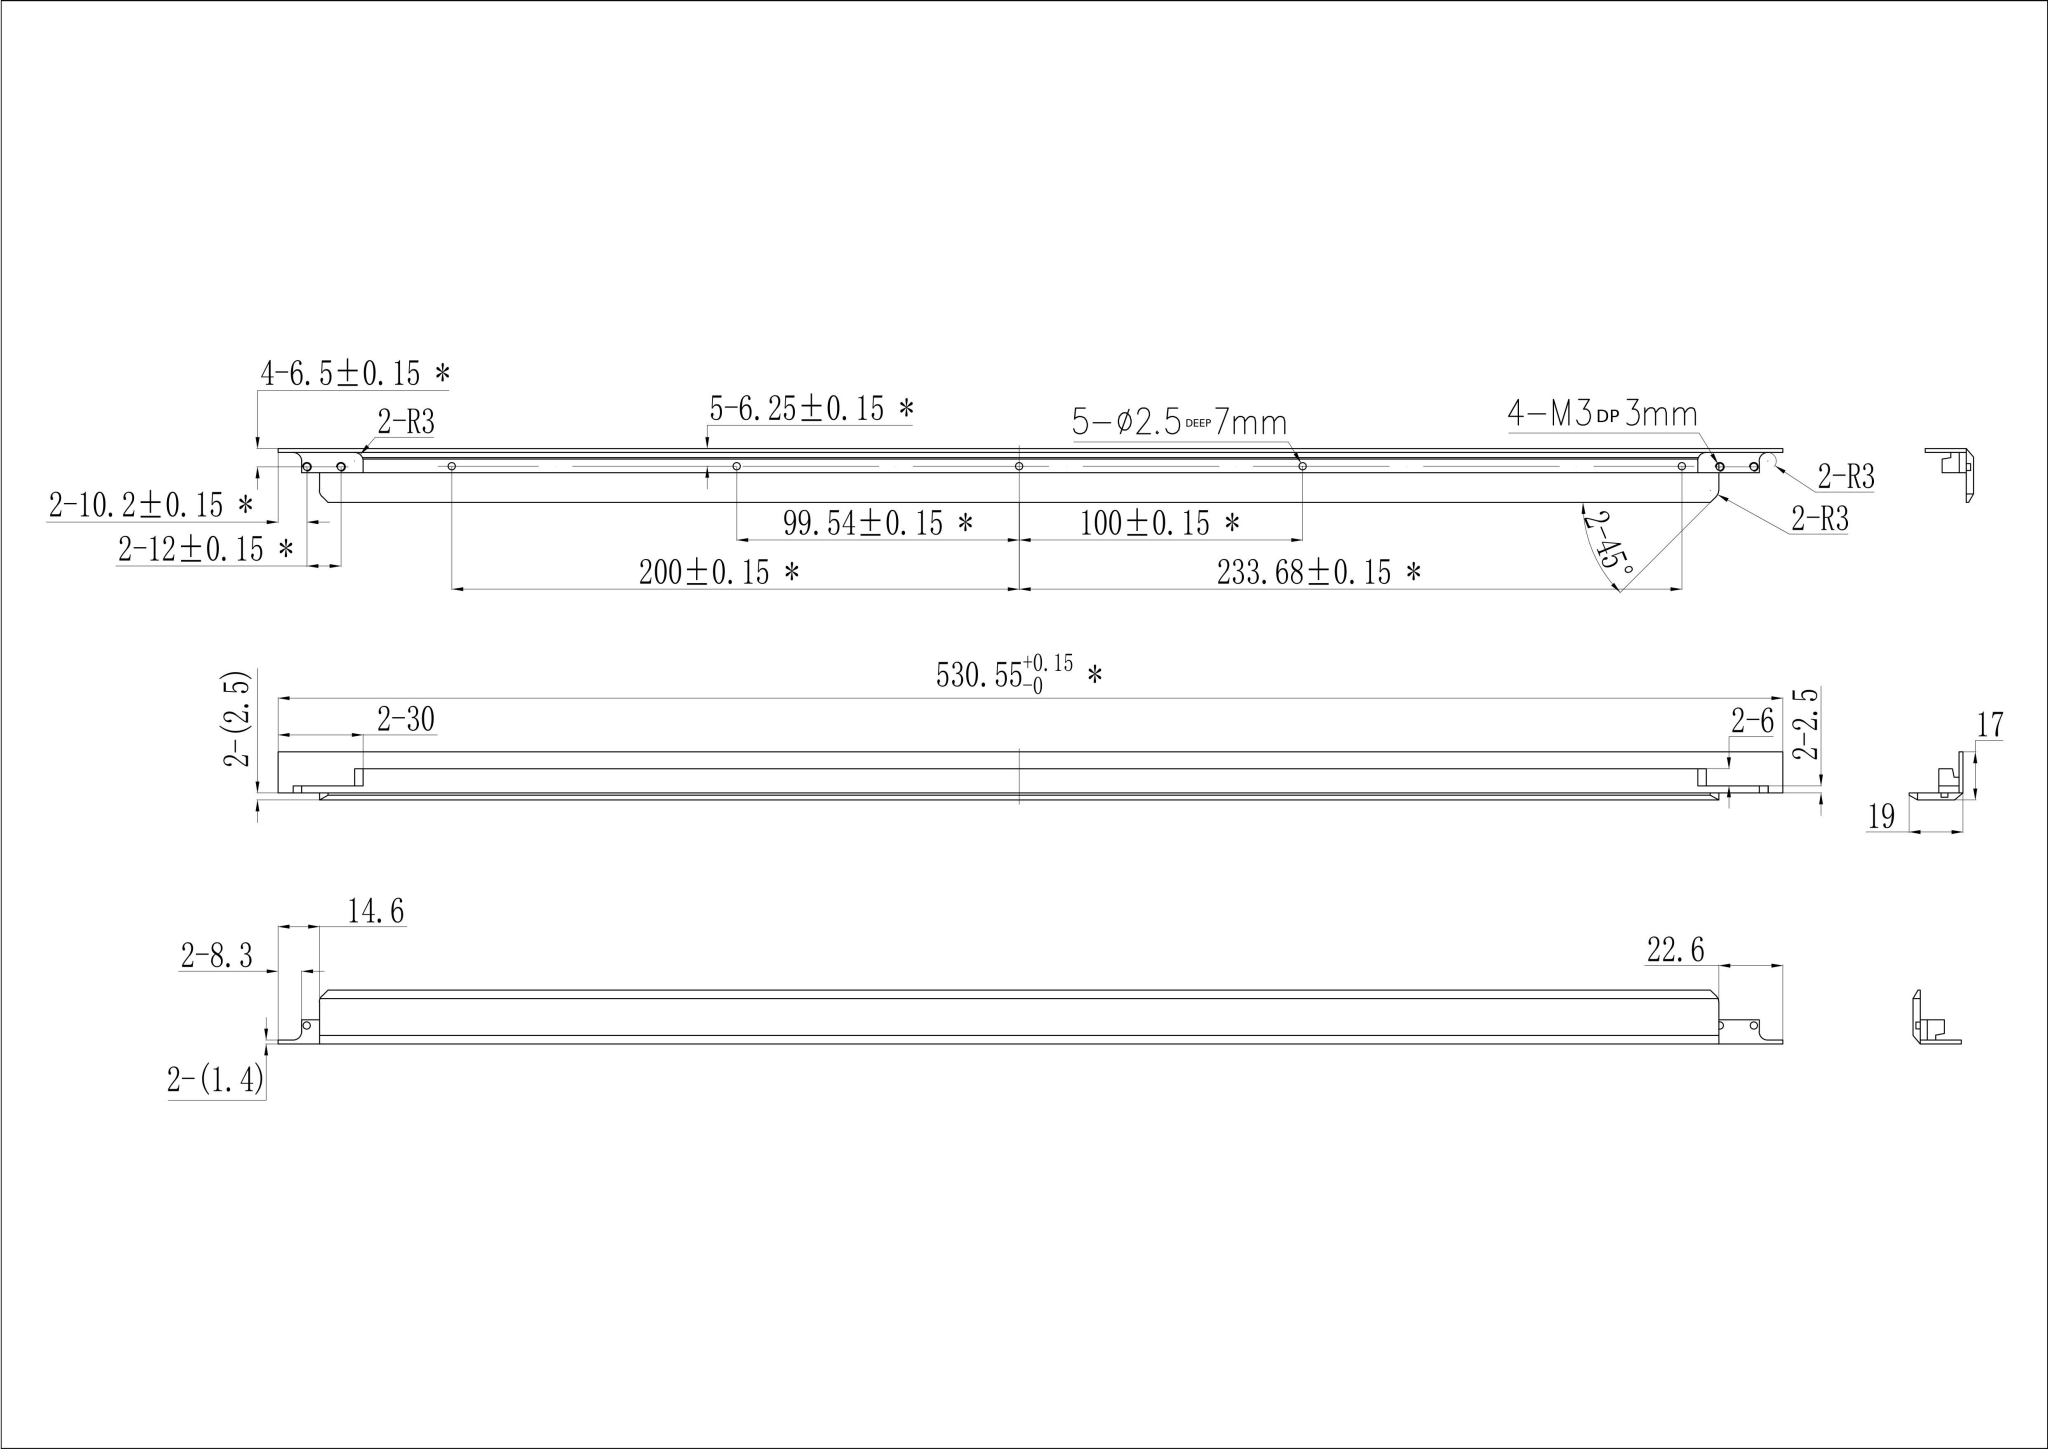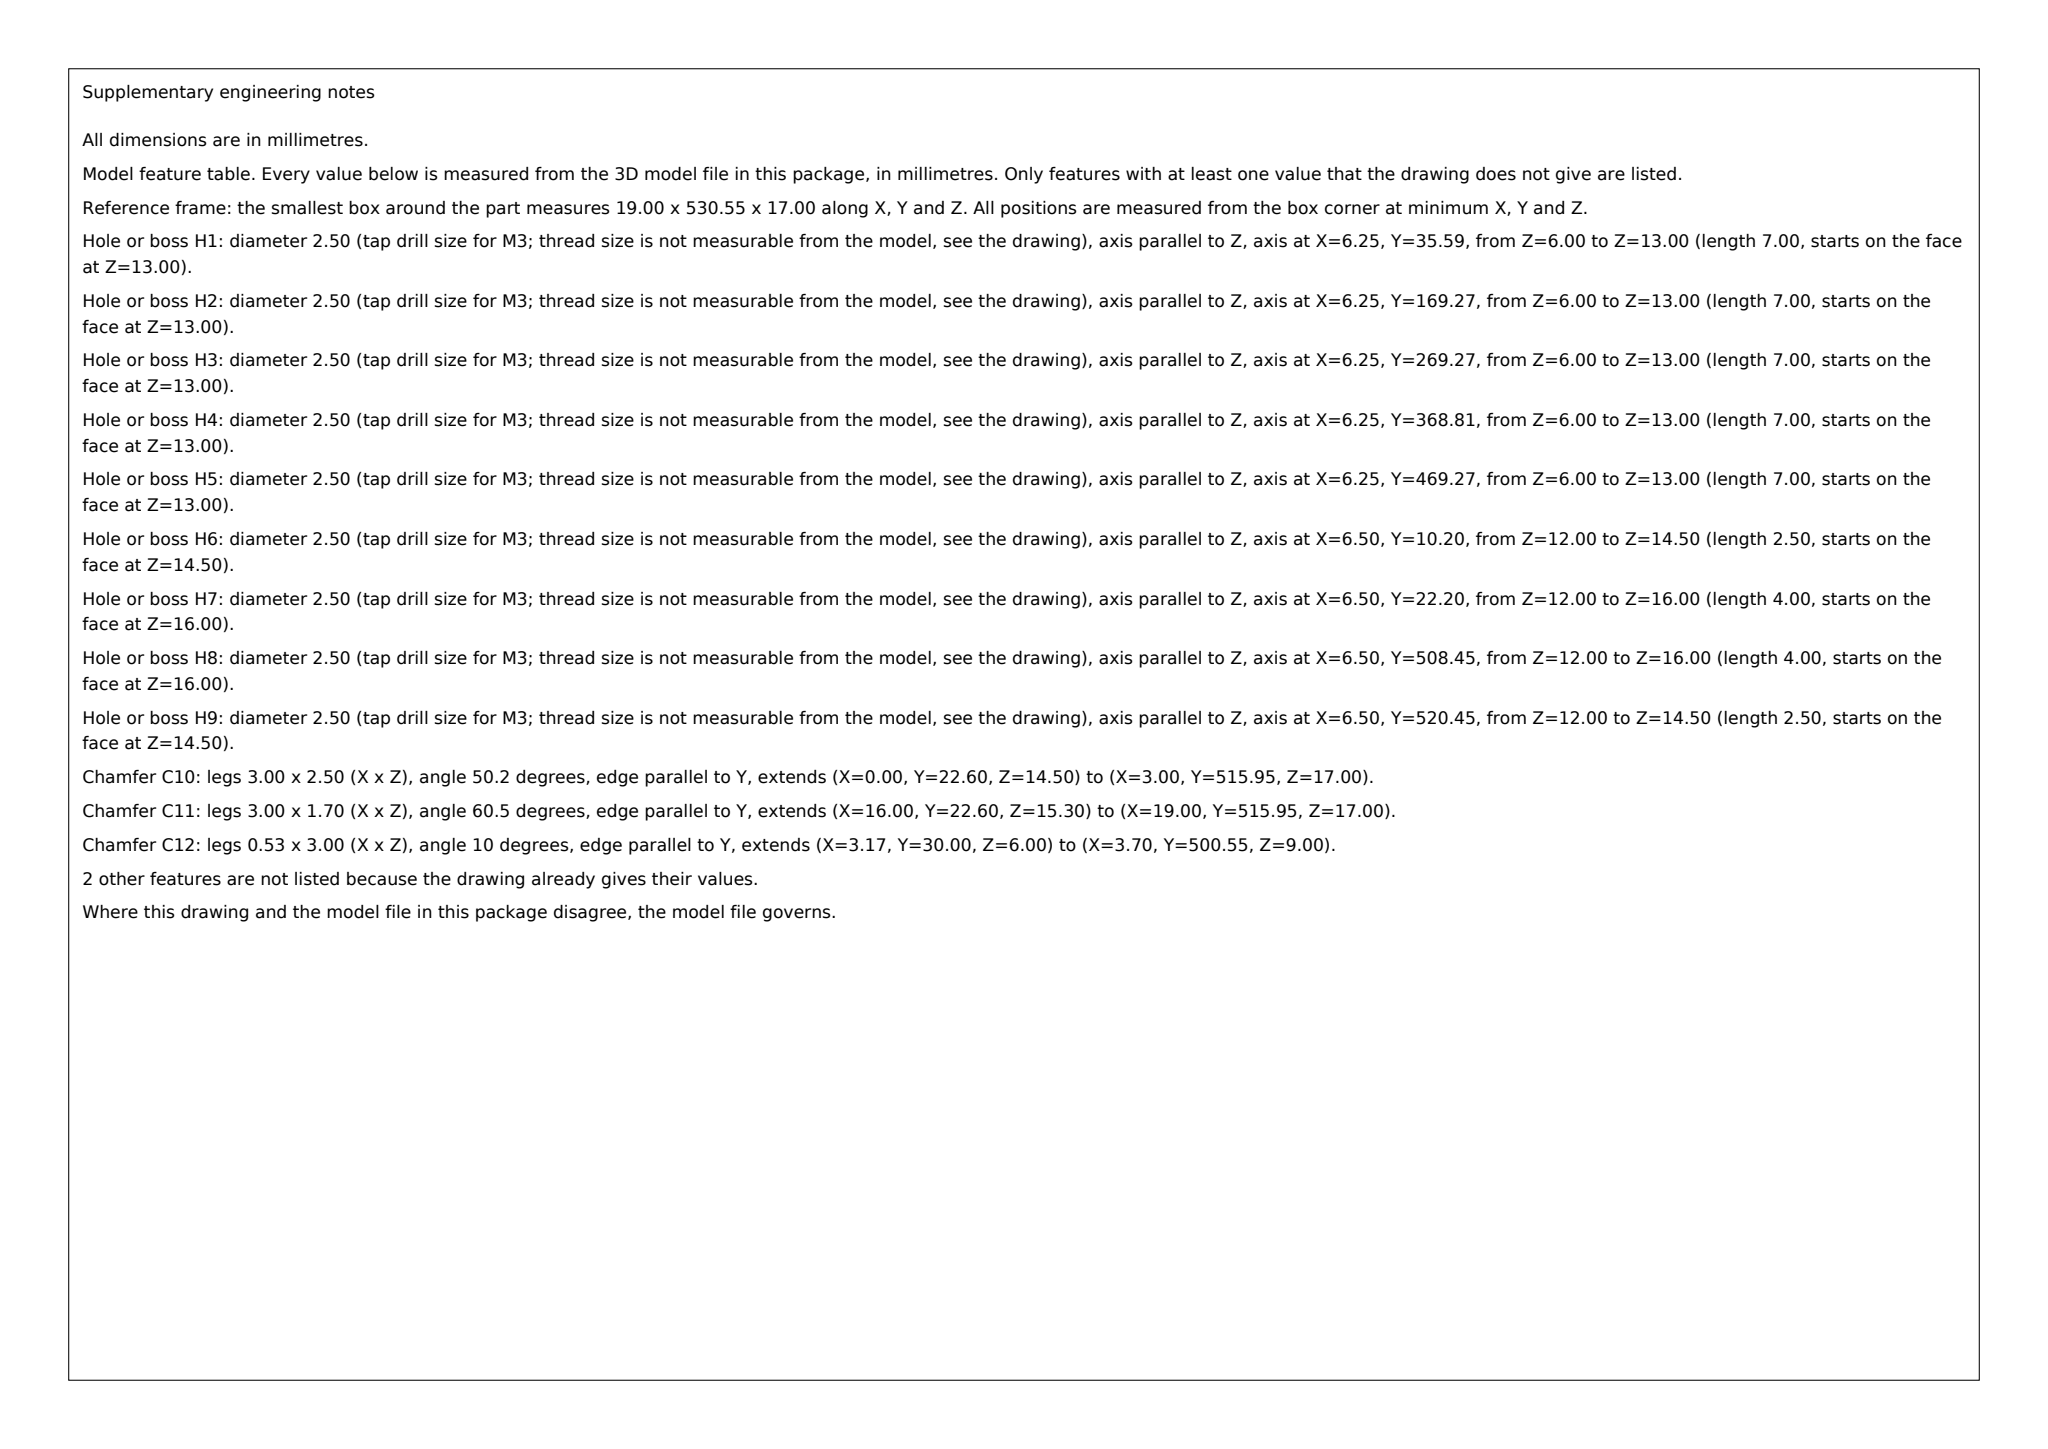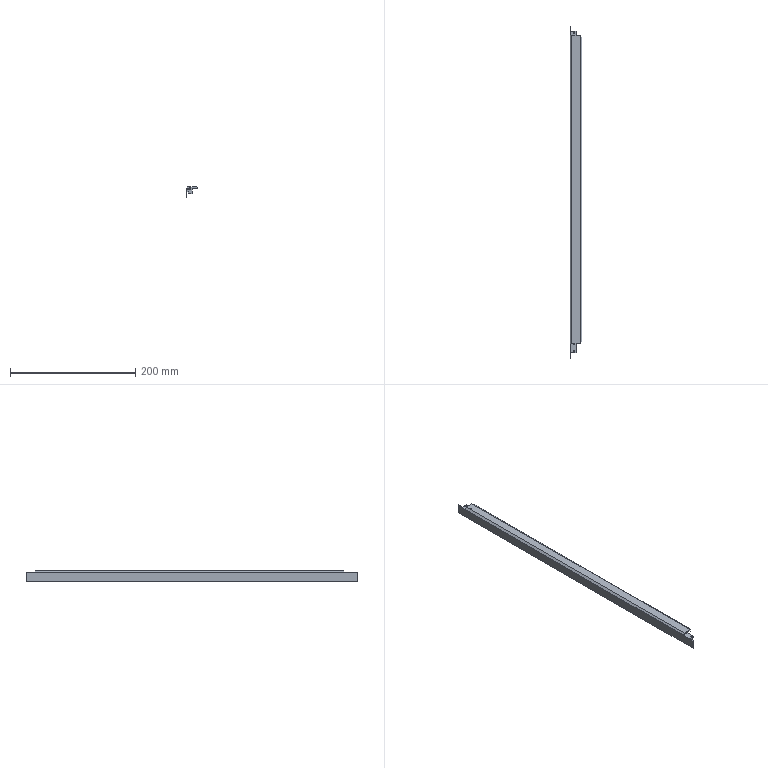Part | SolidWorks | mm | 1 solid | 51 faces | box 19 x 530.55 x 17 mm | volume 61264 mm3 | plane 33 | cylinder 18 | commonest cylinder face diameters 2.5 x18